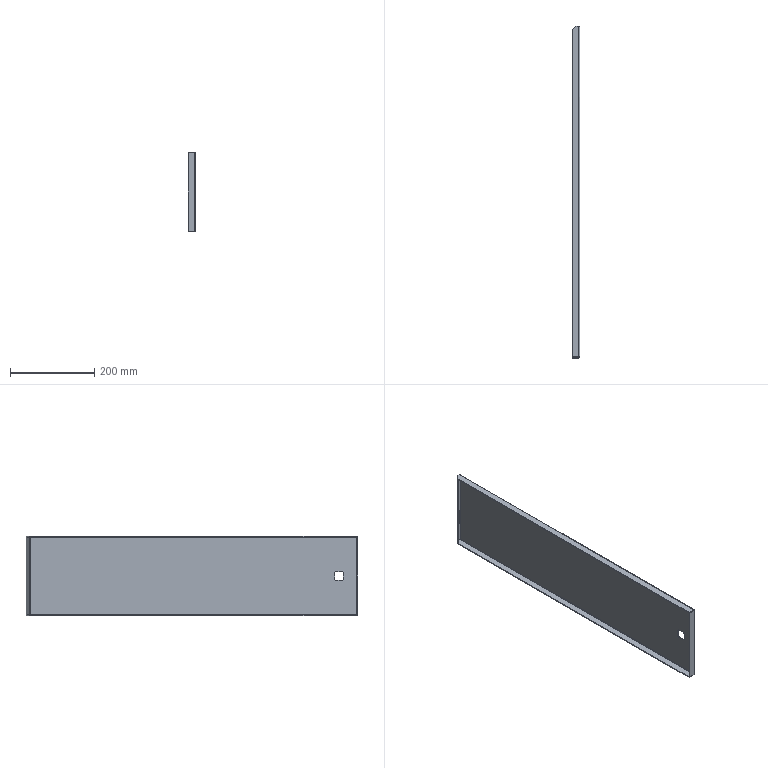Component | SolidWorks | FrontUpperDoor.2-1 | 1 solid | 67 faces | volume 358725 mm3 | plane 49 | cylinder 14 | spline 4 | commonest cylinder face diameters 6 x9 2 x5